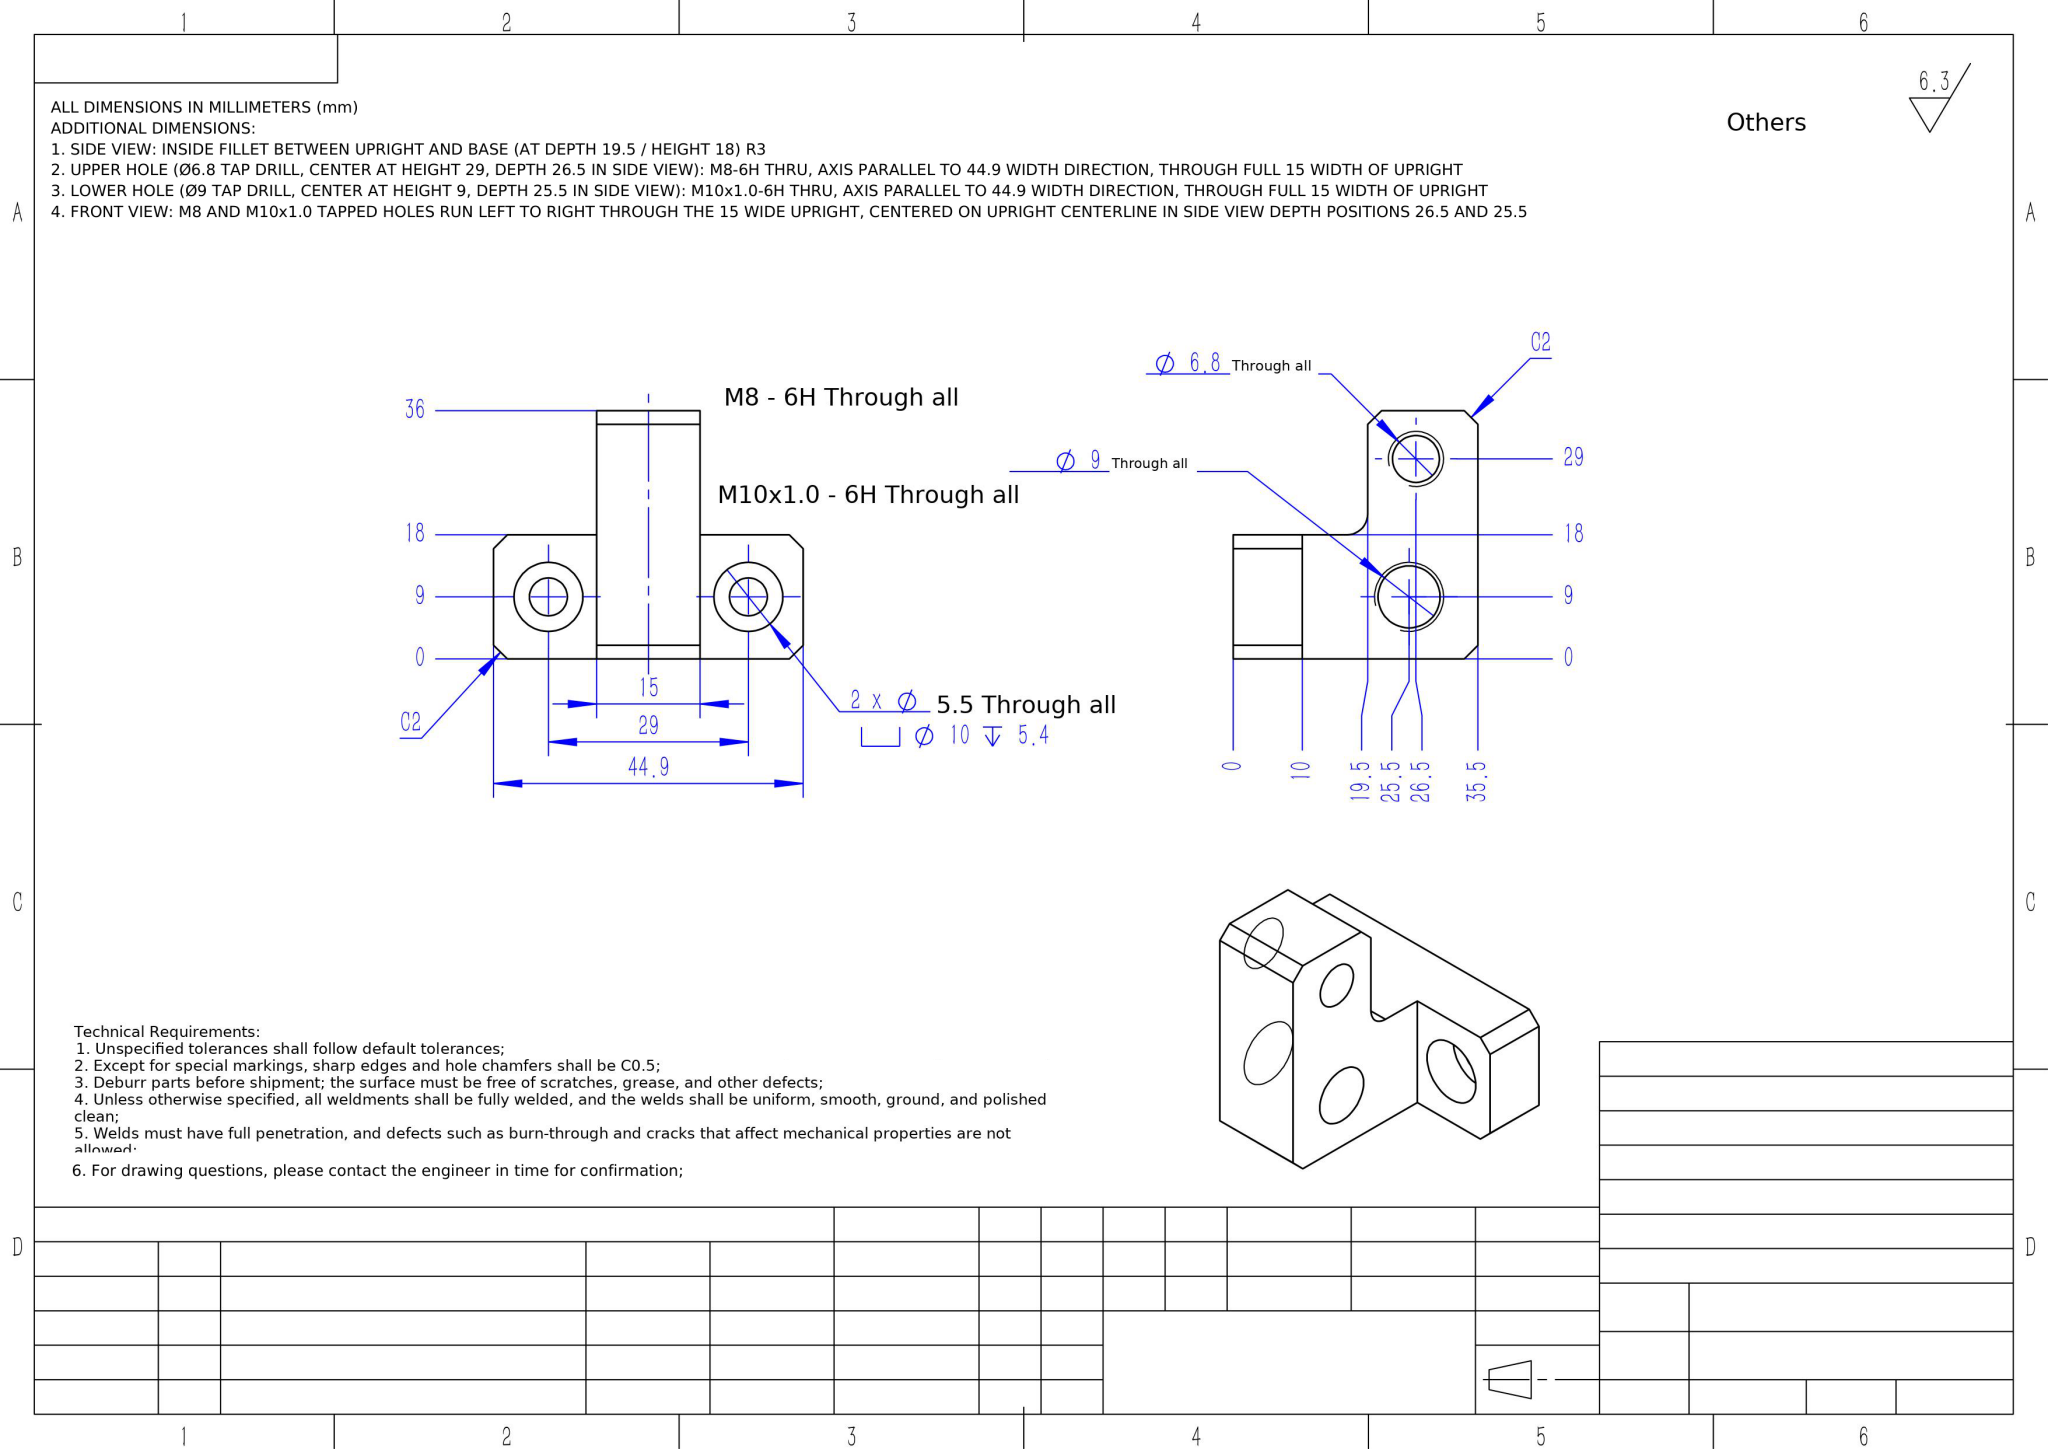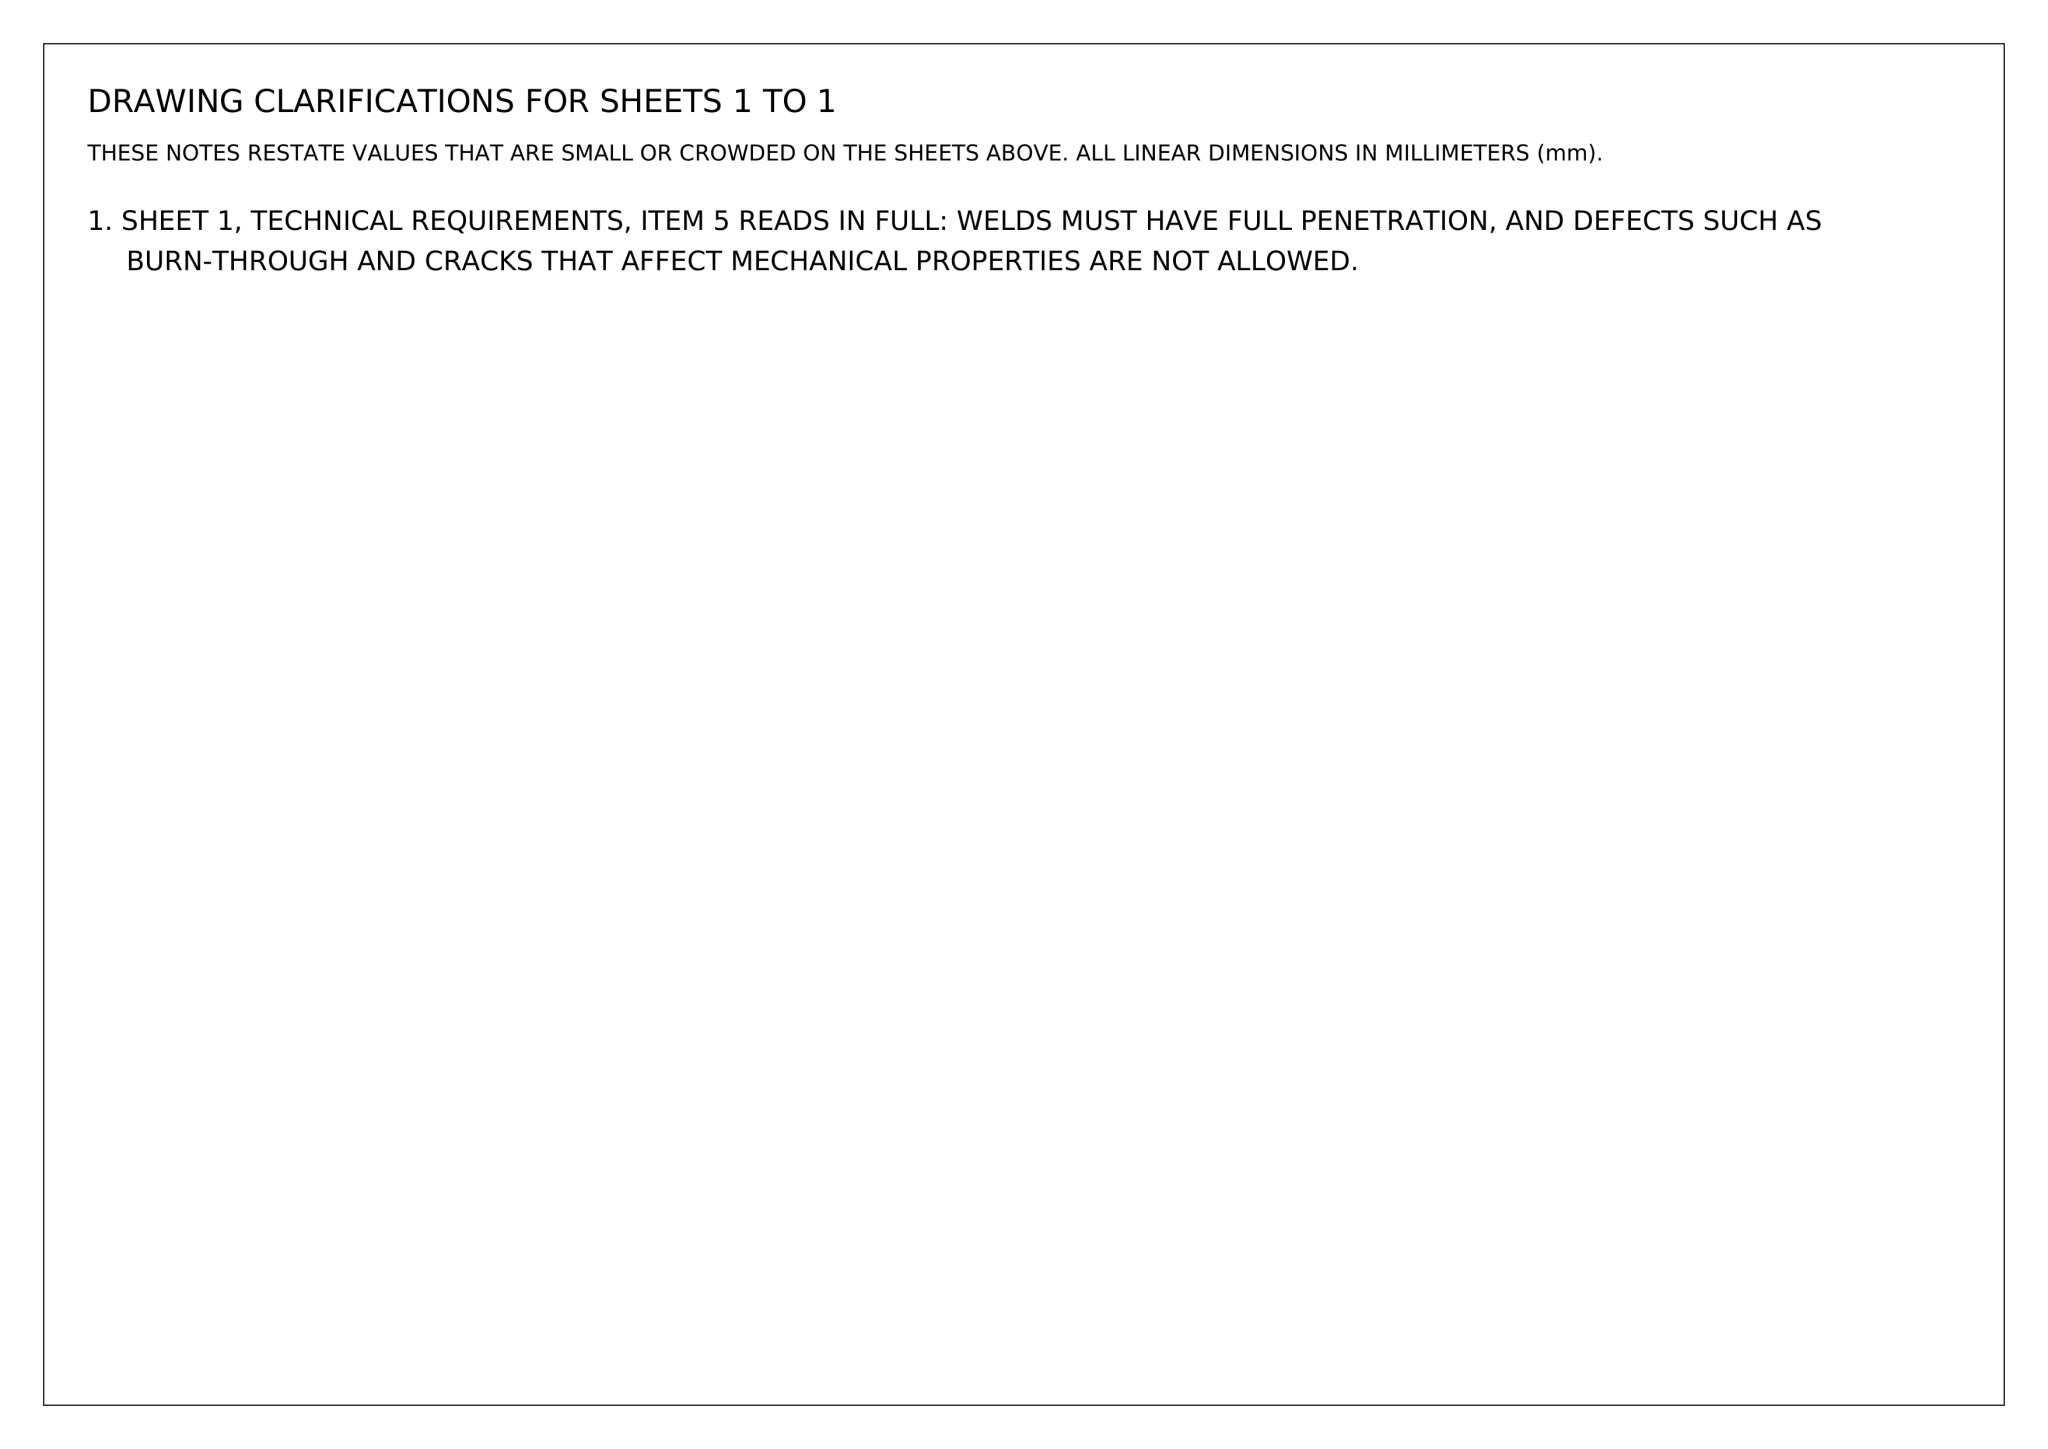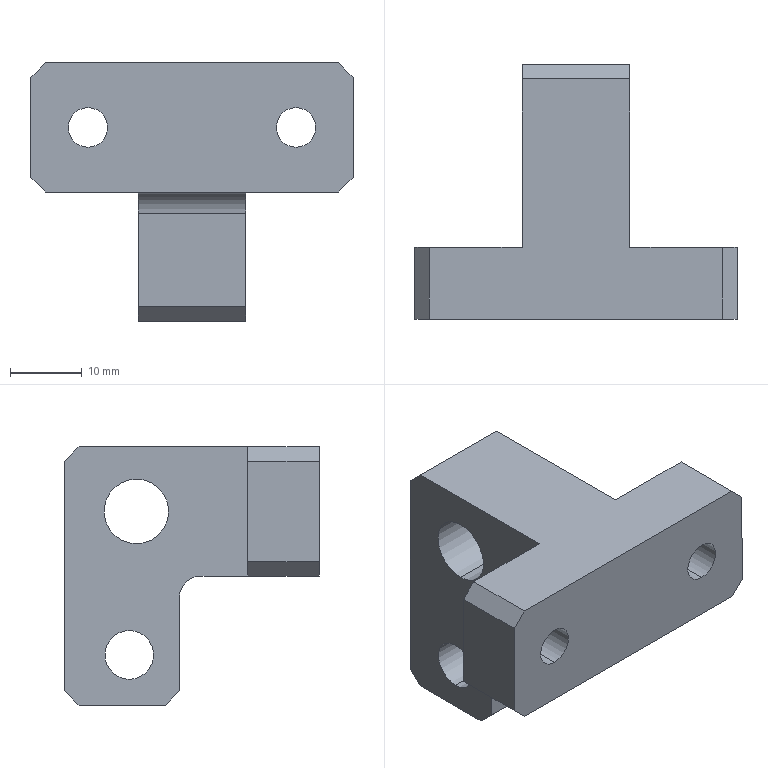Part | NX | mm | 1 solid | 34 faces | box 44.9 x 35.5 x 36 mm | volume 16580 mm3 | plane 21 | cylinder 13 | commonest cylinder face diameters 10 x4 5.5 x4 9 x2 6.8 x2 6 x1